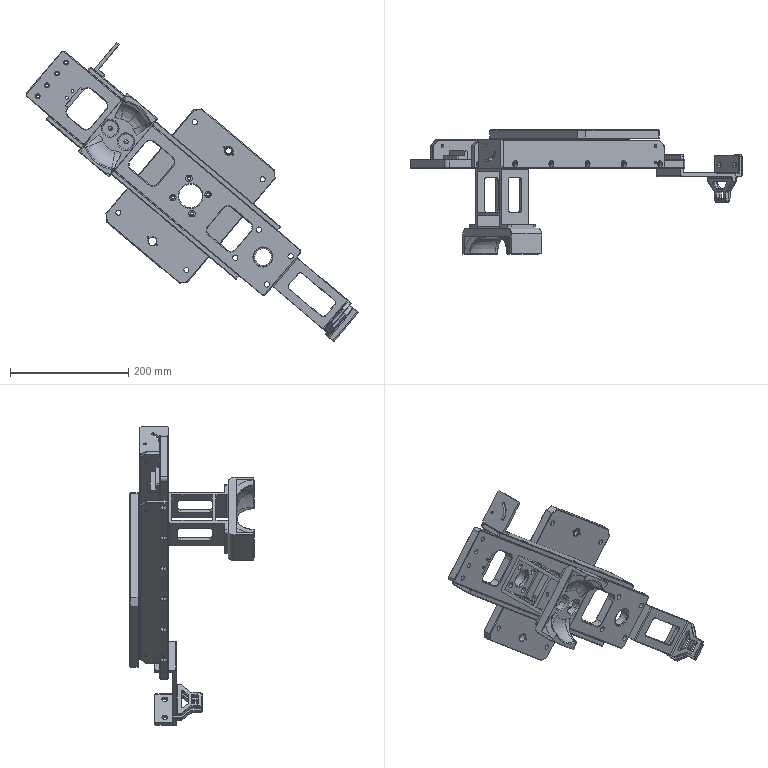Assembly | SolidWorks | mm | 12 component files | 12 solids | 1124 faces | box 560.99 x 210.08 x 504.34 mm | volume 1981357 mm3 | cylinder 402 | plane 396 | cone 260 | spline 44 | torus 15 | sphere 7 | commonest cylinder face diameters 4 x53 5 x52 6.6 x48 11 x40 10 x34 9.5 x24 1 x17 6.8 x16
Bill of materials:
01GripperConnectionPlate | 1 | Aviation Aluminum-7075 | Flat rectangular plate with chamfered corners, a large central round hole inside a shallow square recess, and several smaller holes near the edges.
02GripperBasePlate | 1 | Aviation Aluminum-7075 | Long narrow flat bar with a row of cutouts: rounded-square windows alternating with round holes that each have four small holes around them. There are also small holes along one long edge face.
03LocatingBlock | 1 | Aviation Aluminum-7075 | Square block with rounded corners and a large round bore running through it. Each corner has a small axial hole.
04ReinforcingRib | 2 | Aviation Aluminum-7075 | Long thin flat strip with angled chamfers at two diagonally opposite corners. It has a row of holes along one long edge and a few smaller holes near each end.
05CameraLensMountPlate | 1 | Aviation Aluminum-7075 | Small block with a flat plate portion holding two through holes, a perpendicular rib or flange along one edge, and a rectangular tab sticking out from the opposite side.
06CameraLightSourceMountPlate | 1 | Aviation Aluminum-7075 | L-shaped angle bracket. One leg has two countersunk holes. The other leg has a curved arc slot and a small round hole.
07FixtureBase | 1 | Aviation Aluminum-7075 | Bracket shaped like a box or channel, with base mounting flanges and an internal web. The walls have rounded rectangular windows, and each base flange has a pair of round holes.
08ProfileFixture | 1 | Nylon66 | Rectangular block with a semicircular cradle (saddle) cut into one face and two round through holes. Edges are rounded.
09GripperJawA | 1 | Aviation Aluminum-7075 | Bracket with a joggled (offset) or stepped profile. One plate has two round holes. The other part tapers and has a triangular window and a small rectangular window.
10GripperJawAA | 1 | Aviation Aluminum-7075 | Long offset bracket. One end has a plate with two holes. The other end is a tapered arm with a triangular cutout and a small rectangular cutout. A long side wall has a large rounded rectangular window.
13LocatingSleeve | 1 | 45(Ni) | Flanged cylindrical bushing: a round flange with a cylindrical hub and a central bore. The flange has small axial holes.
Mates:
1. concentric | 02GripperBasePlate-1 face at (-144.488, 197.645, -264.11) dir (0, -1, 0) r 20 | assembly face at (-144.488, 200.645, -264.11) dir (0, -1, 0) r 20
2. coincident | 02GripperBasePlate-1 face at (-144.488, 199.645, -264.11) dir (0, 1, 0) | assembly face at (-144.488, 189.645, -264.11) dir (0, -1, 0)
3. coincident | assembly face at (-351.273, 79.579, 73.355) dir (-0.6441, 0, -0.765) | assembly face at (-351.273, 106.329, 73.355) dir (0.6441, 0, 0.765)
4. concentric | assembly face at (-343.544, 79.579, 82.535) dir (-0.6441, 0, -0.765) r 42 | assembly face at (-354.654, 79.579, 69.339) dir (-0.6441, 0, -0.765) r 37
5. coincident | 02GripperBasePlate-1 face at (-332.746, 149.645, -170.971) dir (-0.6441, 0, -0.765) | assembly face at (-716.509, 164.579, 274.972) dir (0.6441, 0, 0.765)
6. coincident | 02GripperBasePlate-1 face at (-144.488, 164.645, -264.11) dir (0, 1, 0) | assembly face at (-726.17, 164.579, 263.497) dir (0, 1, 0)
7. distance | assembly face at (-299.312, 154.579, -95.886) dir (-0.6441, 0, -0.765) r 3.3 | 02GripperBasePlate-1 face at (-307.475, 144.579, -69.405) dir (-0.765, 0, 0.6441)
8. concentric | assembly face at (-367.085, 79.579, -15.295) dir (-0.6441, 0, -0.765) r 5.75 | assembly face at (-360.383, 79.579, -7.335) dir (-0.6441, 0, -0.765) r 4.188
9. coincident | assembly face at (-716.509, 164.579, 274.972) dir (0.6441, 0, 0.765) | assembly face at (-443.583, 102.763, 49.11) dir (-0.6441, 0, -0.765)
10. parallel | assembly face at (-726.17, 164.579, 263.497) dir (0, 1, 0) | assembly face at (-413.441, 164.579, 84.911) dir (0, 1, 0)
11. parallel | assembly face at (-356.425, 294.579, 67.235) dir (0, 1, 0) | assembly face at (-726.17, 164.579, 263.497) dir (0, 1, 0)
12. coincident | 02GripperBasePlate-1 face at (-144.488, 149.645, -264.11) dir (0, -1, 0) | assembly face at (-103.509, 144.579, -132.63) dir (0, 1, 0)
13. parallel | 02GripperBasePlate-1 face at (-268.34, 149.645, -94.473) dir (0.6441, 0, 0.765) | assembly face at (-80.967, 179.579, -105.856) dir (0.6441, 0, 0.765)
14. width | 02GripperBasePlate-1 face at (-20.635, 149.645, -433.746) dir (0.765, 0, -0.6441) | 02GripperBasePlate-1 face at (-307.475, 144.579, -69.405) dir (-0.765, 0, 0.6441) | assembly face at (-80.967, 179.579, -105.856) dir (-0.765, 0, 0.6441) | assembly face at (-46.543, 179.579, -134.838) dir (0.765, 0, -0.6441)
15. coincident | 02GripperBasePlate-1 face at (-268.34, 149.645, -94.473) dir (0.6441, 0, 0.765) | assembly face at (-90.628, 144.579, -117.33) dir (-0.6441, 0, -0.765)
16. coincident | 02GripperBasePlate-1 face at (-144.488, 149.645, -264.11) dir (0, -1, 0) | assembly face at (-209.477, 149.645, -151.876) dir (0, 1, 0)
17. concentric | 02GripperBasePlate-1 face at (-266.884, 164.646, -161.061) dir (0, -1, 0) r 16 | assembly face at (-266.884, 149.645, -161.061) dir (0, 1, 0) r 16
18. parallel | 02GripperBasePlate-1 face at (-213.903, 149.644, -166.45) dir (0.765, 0, -0.6441) | assembly face at (-209.477, 125.145, -151.876) dir (0.765, 0, -0.6441)
19. coincident | 02GripperBasePlate-1 face at (-268.34, 149.645, -94.473) dir (0.6441, 0, 0.765) | 04ReinforcingRib-1 face at (2.462, 149.645, -322.469) dir (-0.6441, 0, -0.765)
20. coincident | 02GripperBasePlate-1 face at (-144.488, 149.645, -264.11) dir (0, -1, 0) | 04ReinforcingRib-1 face at (7.614, 149.645, -316.349) dir (0, -1, 0)
21. coincident | 02GripperBasePlate-1 face at (-332.746, 149.645, -170.971) dir (-0.6441, 0, -0.765) | 04ReinforcingRib-3 face at (-383.235, 149.645, -128.463) dir (0.6441, 0, 0.765)
22. coincident | 02GripperBasePlate-1 face at (-144.488, 149.645, -264.11) dir (0, -1, 0) | 04ReinforcingRib-3 face at (-388.387, 149.645, -134.583) dir (0, -1, 0)
23. coincident | 04ReinforcingRib-1 face at (7.614, 149.645, -316.349) dir (0.765, 0, -0.6441) | 04ReinforcingRib-3 face at (-67.096, 149.645, -405.087) dir (0.765, 0, -0.6441)
24. coincident | assembly face at (-250.144, 68.645, -91.492) dir (0.6441, 0, 0.765) | assembly face at (-168.291, -163.545, -160.406) dir (-0.6441, 0, -0.765)
25. concentric | assembly face at (-214.873, 80.645, -130.338) dir (0.6441, 0, 0.765) r 3.324 | assembly face at (-200.06, 80.645, -112.744) dir (0.6441, 0, 0.765) r 7.5
26. concentric | assembly face at (-245.473, 80.645, -104.576) dir (0.6441, 0, 0.765) r 3.324 | assembly face at (-230.659, 80.645, -86.981) dir (0.6441, 0, 0.765) r 7.5
27. concentric | 08ProfileFixture-1 face at (-253.497, 48.645, -172.332) dir (0, 1, 0) r 2.1 | assembly face at (-251.585, 41.695, -173.942) dir (0, -1, 0) r 4.5
28. coincident | 02GripperBasePlate-1 face at (-144.488, 149.645, -264.11) dir (0, -1, 0) | 07FixtureBase-1 face at (-311.731, 149.645, -167.748) dir (0, 1, 0)
29. concentric | 02GripperBasePlate-1 face at (-144.488, 149.644, -264.11) dir (0, 1, 0) r 20 | 03LocatingBlock-1 face at (-144.488, 204.645, -264.11) dir (0, -1, 0) r 20
30. concentric | 02GripperBasePlate-1 face at (-141.923, 149.645, -294) dir (0, -1, 0) r 3.3 | 03LocatingBlock-1 face at (-141.923, 204.645, -294) dir (0, 1, 0) r 2.5
31. coincident | 02GripperBasePlate-1 face at (-144.488, 159.645, -264.11) dir (0, 1, 0) | 03LocatingBlock-1 face at (-147.511, 159.645, -228.884) dir (0, -1, 0)
32. concentric | 03LocatingBlock-1 face at (-144.488, 204.645, -264.11) dir (0, -1, 0) r 20 | 01GripperConnectionPlate-1 face at (-144.488, 214.646, -264.11) dir (0, -1, 0) r 20
33. coincident | 03LocatingBlock-1 face at (-147.511, 204.645, -228.884) dir (0, 1, 0) | 01GripperConnectionPlate-1 face at (-144.488, 204.645, -264.11) dir (0, -1, 0)
34. concentric | 03LocatingBlock-1 face at (-141.923, 204.645, -294) dir (0, 1, 0) r 2.5 | 01GripperConnectionPlate-1 face at (-141.923, 214.645, -294) dir (0, 1, 0) r 5.5
35. concentric | 08ProfileFixture-1 face at (-253.497, 48.645, -172.332) dir (0, 1, 0) r 2.1 | assembly face at (-251.585, 47.3, -173.942) dir (0, -1, 0) r 2.5
36. width | 02GripperBasePlate-1 face at (-20.635, 149.645, -433.746) dir (0.765, 0, -0.6441) | 02GripperBasePlate-1 face at (-424.543, -6.56, -93.684) dir (-0.765, 0, 0.6441) | 04ReinforcingRib-1 face at (-313.677, 149.645, -45.846) dir (-0.765, 0, 0.6441) | 04ReinforcingRib-1 face at (7.614, 149.645, -316.349) dir (0.765, 0, -0.6441)
37. concentric | 08ProfileFixture-1 face at (-253.497, 43.645, -172.332) dir (0, -1, 0) r 13 | assembly face at (-253.497, 50.895, -172.332) dir (0, -1, 0) r 6.5
38. coincident | 08ProfileFixture-1 face at (-266.884, 33.645, -161.061) dir (0, -1, 0) | assembly face at (-259.88, 33.645, -176.502) dir (0, -1, 0)
39. coincident | 08ProfileFixture-1 face at (-266.321, 48.645, -189.447) dir (0, 1, 0) | 07FixtureBase-1 face at (-307.867, 48.645, -163.158) dir (0, -1, 0)
40. concentric | 08ProfileFixture-1 face at (-282.48, 48.645, -206.756) dir (0, 1, 0) r 3.4 | 07FixtureBase-1 face at (-282.48, 149.646, -206.756) dir (0, -1, 0) r 4.75
41. coincident | 02GripperBasePlate-1 face at (-144.488, 164.645, -264.11) dir (0, 1, 0) | 05CameraLensMountPlate-1 face at (-367.738, 164.645, -102.294) dir (0, -1, 0)
42. coincident | 02GripperBasePlate-1 face at (-343.382, 164.645, -96.655) dir (0.765, 0, -0.6441) | 05CameraLensMountPlate-1 face at (-343.382, 164.695, -96.655) dir (-0.765, 0, 0.6441)
43. coincident | 02GripperBasePlate-1 face at (-330.501, 177.145, -81.355) dir (-0.6441, 0, -0.765) | 05CameraLensMountPlate-1 face at (-330.501, 179.745, -81.355) dir (0.6441, 0, 0.765)
44. coincident | 04ReinforcingRib-1 face at (7.614, 149.645, -316.349) dir (0.6441, 0, 0.765) | 06CameraLightSourceMountPlate-1 face at (-303.732, 149.645, -54.218) dir (-0.6441, 0, -0.765)
45. parallel | 04ReinforcingRib-1 face at (-313.677, 149.645, -45.846) dir (-0.765, 0, 0.6441) | 06CameraLightSourceMountPlate-1 face at (-272.935, 173.645, -40.93) dir (0.765, 0, -0.6441)
46. concentric | 04ReinforcingRib-1 face at (-298.377, 187.645, -58.727) dir (0.6441, 0, 0.765) r 2.5 | 06CameraLightSourceMountPlate-1 face at (-295.157, 187.645, -54.902) dir (0.6441, 0, 0.765) r 3.3
47. coincident | 01GripperConnectionPlate-1 face at (-80.082, 209.645, -187.612) dir (0, 1, 0) | 13LocatingSleeve-1 face at (-80.082, 209.645, -187.612) dir (0, -1, 0)
48. concentric | 01GripperConnectionPlate-1 face at (-80.082, 199.644, -187.612) dir (0, 1, 0) r 7 | 13LocatingSleeve-1 face at (-80.082, 209.645, -187.612) dir (0, 1, 0) r 13.5
49. concentric | 01GripperConnectionPlate-1 face at (-72.432, 209.645, -194.052) dir (0, 1, 0) r 1.25 | 13LocatingSleeve-1 face at (-72.432, 214.645, -194.052) dir (0, 1, 0) r 3
50. coincident | 09GripperJawA-1 face at (124.281, 142.645, -448.562) dir (-0.765, 0, 0.6441) | 10GripperJawAA-5 face at (85.913, 142.645, -494.134) dir (0.765, 0, -0.6441)
51. coincident | 02GripperBasePlate-1 face at (-20.635, 149.645, -433.746) dir (0.765, 0, -0.6441) | 10GripperJawAA-5 face at (-6.191, 135.645, -416.59) dir (-0.765, 0, 0.6441)
52. coincident | 09GripperJawA-1 face at (124.281, 92.645, -448.562) dir (0, -1, 0) | 10GripperJawAA-5 face at (85.913, 92.645, -494.134) dir (0, -1, 0)
53. distance | 10GripperJawAA-5 face at (-6.191, 172.645, -416.59) dir (0, 1, 0) | 02GripperBasePlate-1 face at (-144.488, 149.645, -264.11) dir (0, -1, 0)